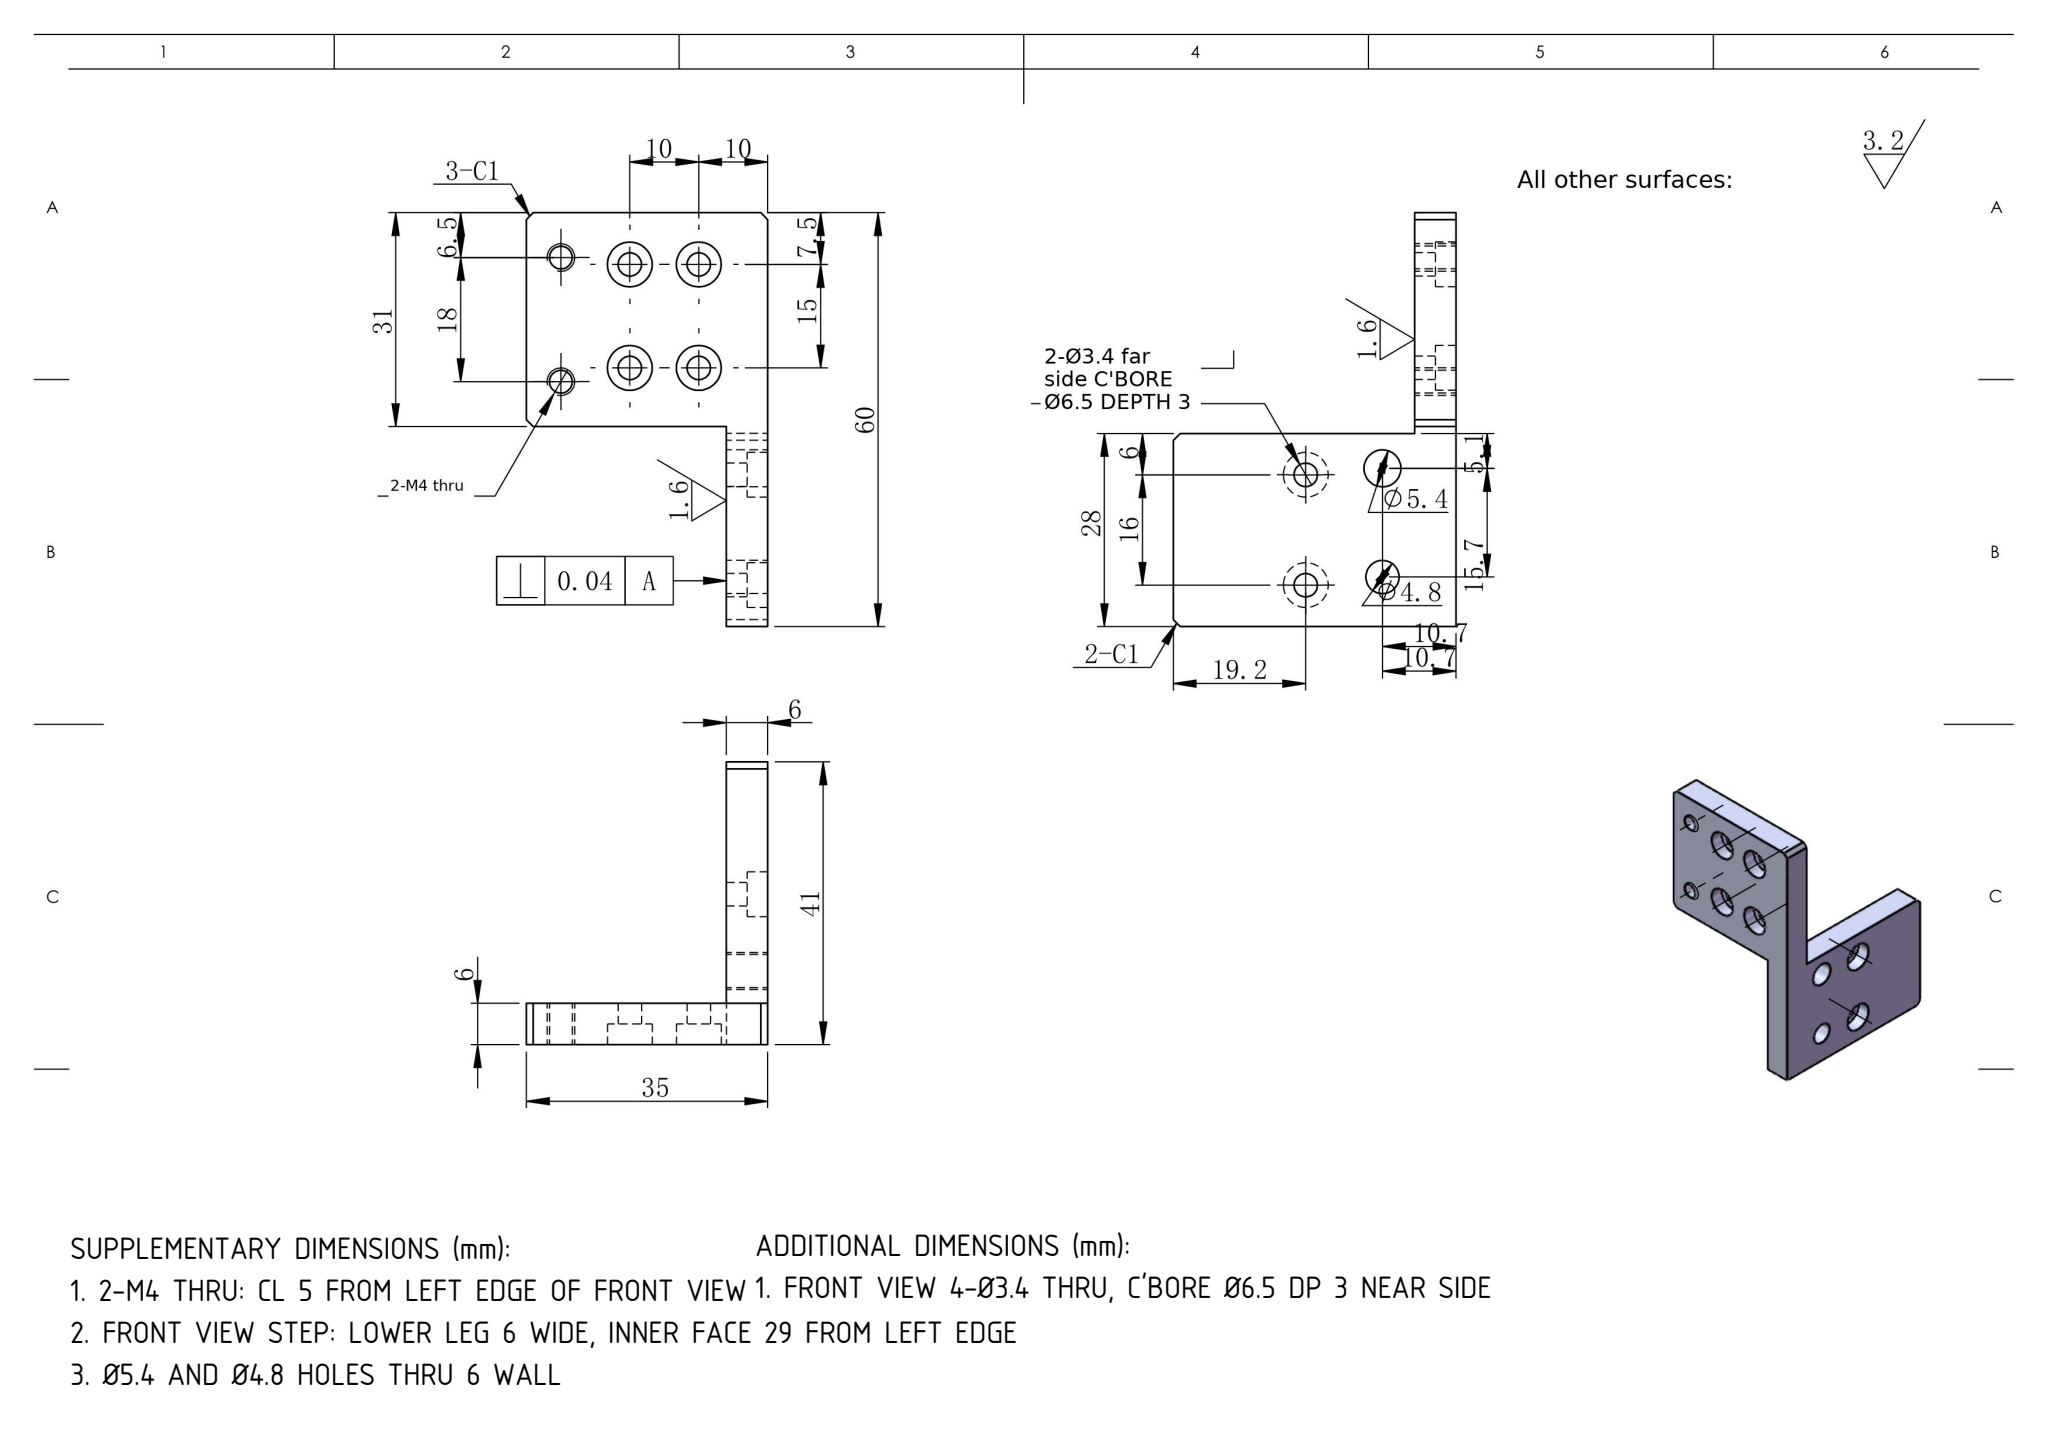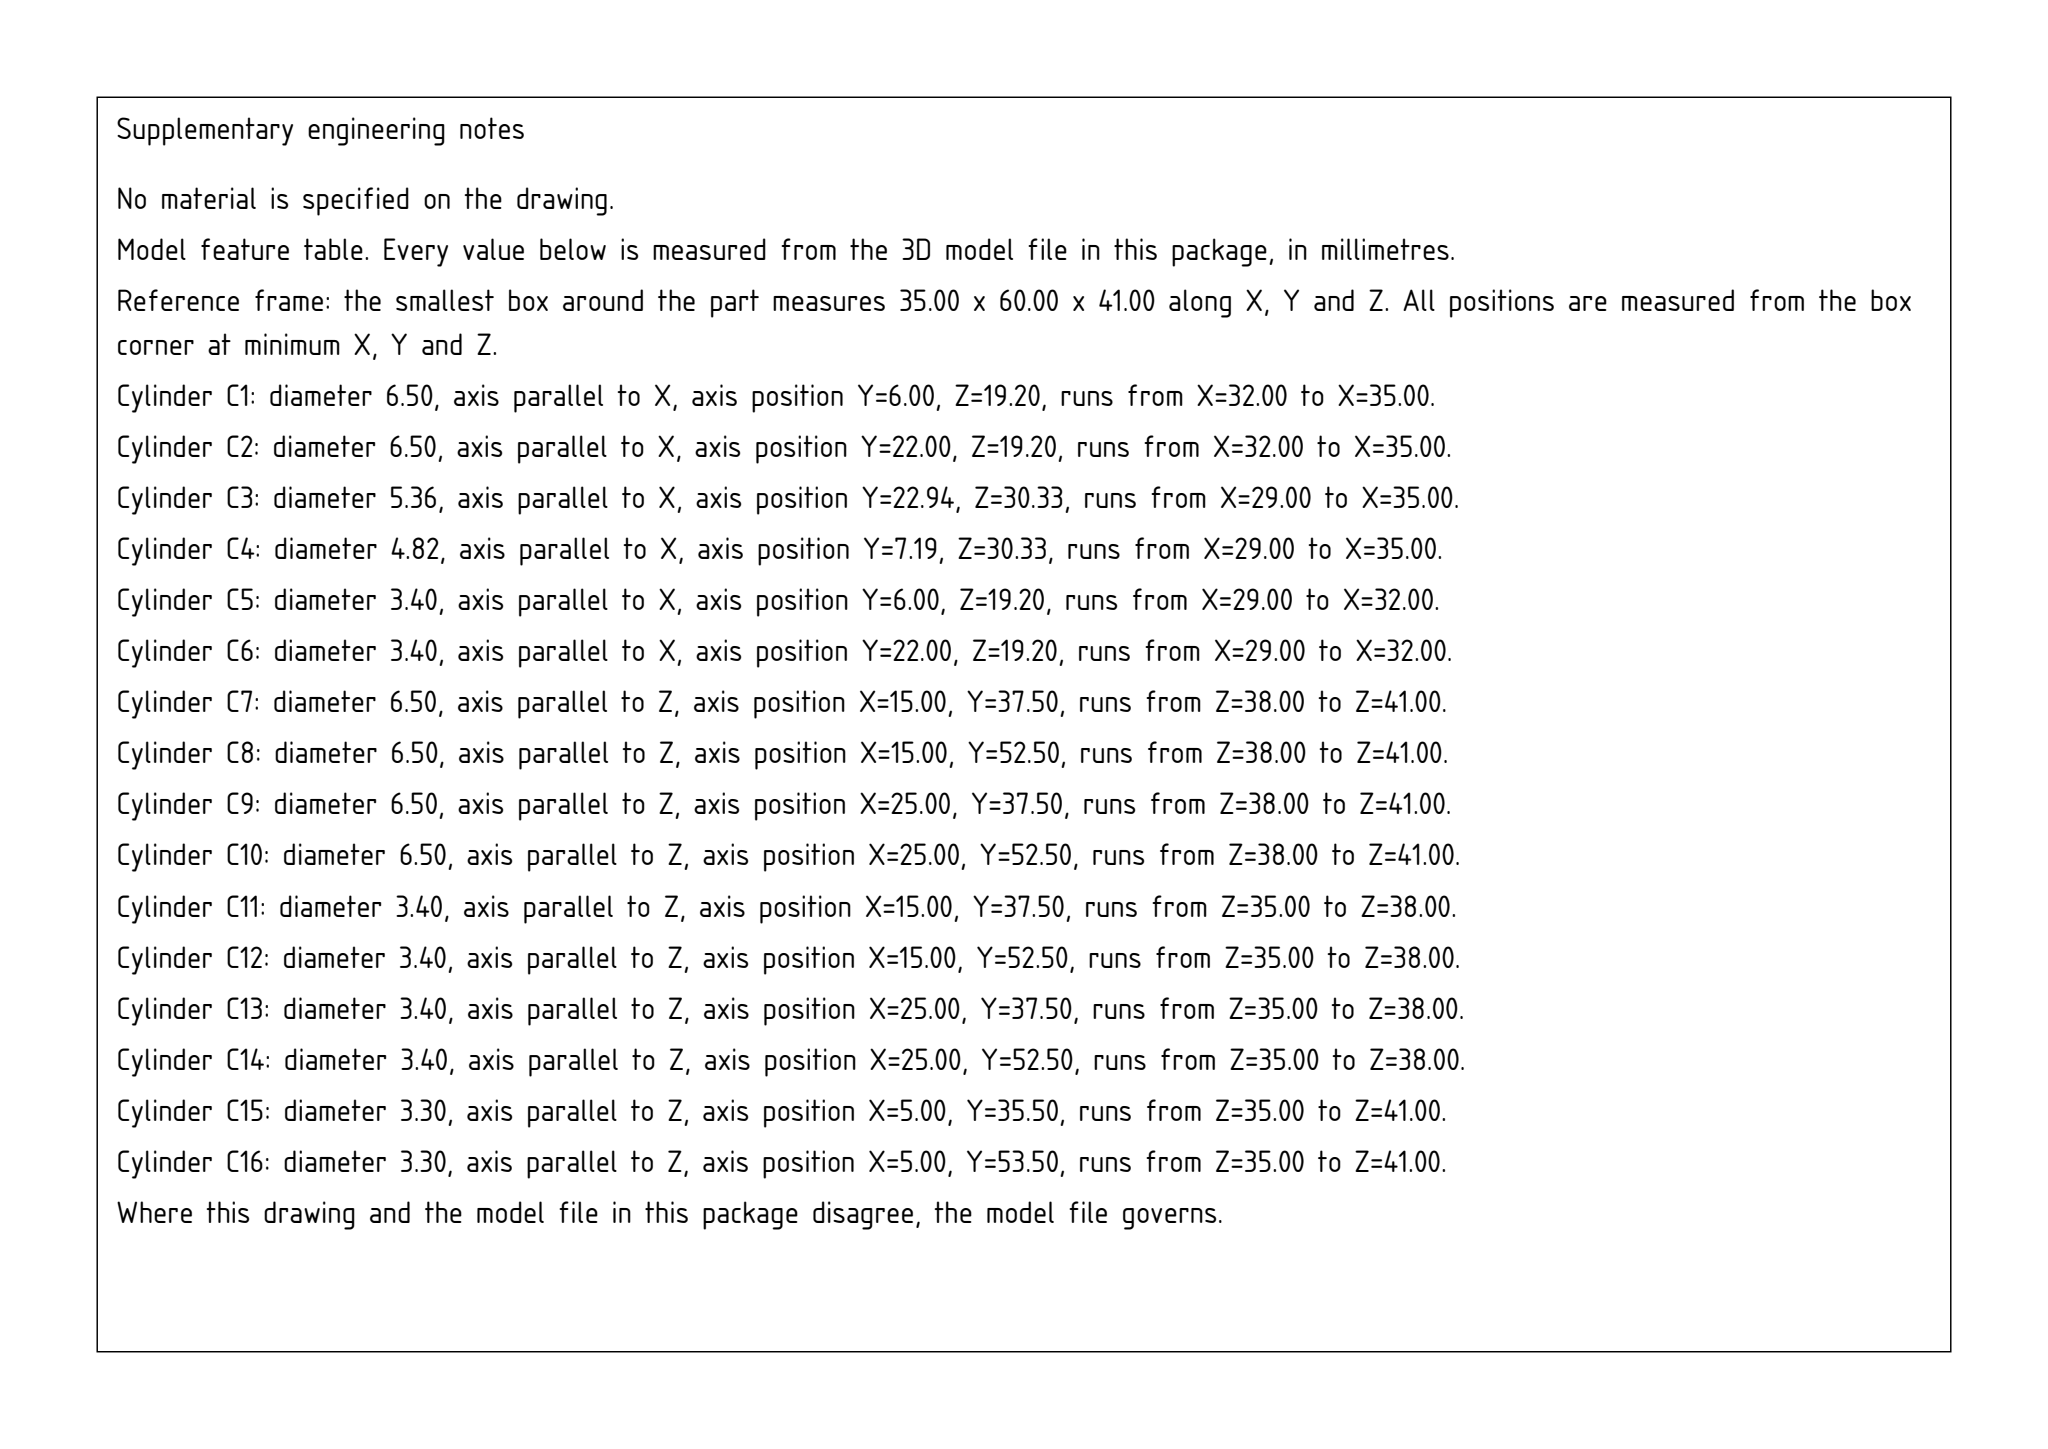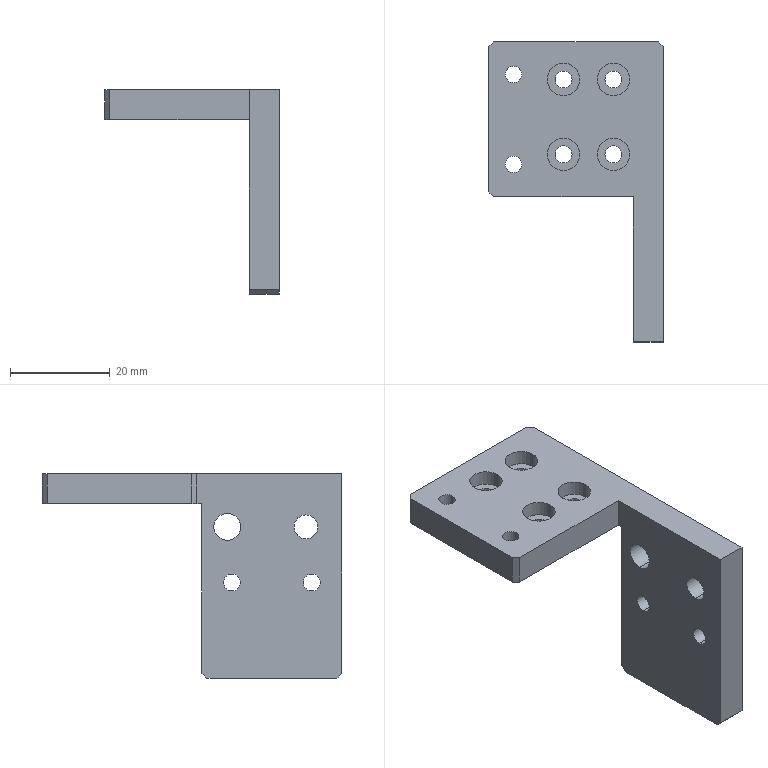Part | SolidWorks | mm | 1 solid | 53 faces | box 35 x 60 x 41 mm | volume 12311 mm3 | cylinder 32 | plane 21 | commonest cylinder face diameters 6.5 x12 3.4 x12 3.3 x4 5.358 x2 4.812 x2
build123d program:
from build123d import *

# Parameters (mm, degrees)
SKETCH1_W                                       = 35
SKETCH1_H                                       = 60
EXTRUDE1_DEPTH                                  = 6
M3_HEX_SOCKET_HEAD_CAP_SCREW_CBORE1_D           = 3.4
M3_HEX_SOCKET_HEAD_CAP_SCREW_CBORE1_CBORE_D     = 6.5
M3_HEX_SOCKET_HEAD_CAP_SCREW_CBORE1_CBORE_DEPTH = 3
SKETCH5_W                                       = 6
SKETCH5_H                                       = 28
EXTRUDE2_DEPTH                                  = 35
SKETCH6_W                                       = 29
SKETCH6_H                                       = 29
CUT_EXTRUDE1_DEPTH                              = 78.782
CHAMFER1_SIZE                                   = 1
M4_TAPPED_HOLE1_D                               = 3.3
M3_HEX_SOCKET_HEAD_CAP_SCREW_CBORE2_D           = 3.4
M3_HEX_SOCKET_HEAD_CAP_SCREW_CBORE2_CBORE_D     = 6.5
M3_HEX_SOCKET_HEAD_CAP_SCREW_CBORE2_CBORE_DEPTH = 3
CHAMFER2_SIZE                                   = 1
SKETCH11_R                                      = 2.679
SKETCH11_R_2                                    = 2.406
CUT_EXTRUDE2_DEPTH                              = 10


with BuildPart() as part:
    # Sketch1 → Extrude1 (new body)
    with BuildSketch(Plane.XY):
        with Locations((17.5, 30)):
            Rectangle(SKETCH1_W, SKETCH1_H)
    extrude(amount=EXTRUDE1_DEPTH)

    # M3 Hex Socket Head Cap Screw CBORE1 (through all)
    with Locations(Plane.XY.offset(6)):
        with Locations((15, 52.5), (25, 52.5), (25, 37.5), (15, 37.5)):
            CounterBoreHole(M3_HEX_SOCKET_HEAD_CAP_SCREW_CBORE1_D / 2, M3_HEX_SOCKET_HEAD_CAP_SCREW_CBORE1_CBORE_D / 2, M3_HEX_SOCKET_HEAD_CAP_SCREW_CBORE1_CBORE_DEPTH)

    # Sketch5 → Extrude2 (add)
    with BuildSketch(Plane(origin=(0, 0, 0), x_dir=(-1, 0, 0), z_dir=(0, 0, -1))):
        with Locations((-32, 14)):
            Rectangle(SKETCH5_W, SKETCH5_H)
    extrude(amount=EXTRUDE2_DEPTH)

    # Sketch6 → Cut-Extrude1 (cut, through all)
    with BuildSketch(Plane(origin=(0, 0, 0), x_dir=(-1, 0, 0), z_dir=(0, 0, -1))):
        with Locations((-14.5, 14.5)):
            Rectangle(SKETCH6_W, SKETCH6_H)
    extrude(amount=-CUT_EXTRUDE1_DEPTH, mode=Mode.SUBTRACT)

    # Chamfer1
    chamfer1_edges = [part.edges().sort_by_distance(p)[0] for p in [
        (0, 29, 3),
        (0, 60, 3),
        (35, 60, 3),
    ]]
    chamfer(chamfer1_edges, length=CHAMFER1_SIZE)

    # M4 Tapped Hole1 (through all)
    with Locations(Plane.XY.offset(6)):
        with Locations((5, 53.5), (5, 35.5)):
            Hole(M4_TAPPED_HOLE1_D / 2)

    # M3 Hex Socket Head Cap Screw CBORE2 (through all)
    with Locations(Plane(origin=(35, 0, 0), x_dir=(0, 0, -1), z_dir=(1, 0, 0))):
        with Locations((15.8, 22), (15.8, 6)):
            CounterBoreHole(M3_HEX_SOCKET_HEAD_CAP_SCREW_CBORE2_D / 2, M3_HEX_SOCKET_HEAD_CAP_SCREW_CBORE2_CBORE_D / 2, M3_HEX_SOCKET_HEAD_CAP_SCREW_CBORE2_CBORE_DEPTH)

    # Chamfer2
    chamfer2_edges = [part.edges().sort_by_distance(p)[0] for p in [
        (32, 0, -35),
        (32, 28, -35),
    ]]
    chamfer(chamfer2_edges, length=CHAMFER2_SIZE)

    # Sketch11 → Cut-Extrude2 (cut)
    with BuildSketch(Plane(origin=(35, 0, 0), x_dir=(0, 0, -1), z_dir=(1, 0, 0))):
        with Locations((4.667, 22.939)):
            Circle(SKETCH11_R)
        with Locations((4.667, 7.19)):
            Circle(SKETCH11_R_2)
    extrude(amount=-CUT_EXTRUDE2_DEPTH, mode=Mode.SUBTRACT)


solid = part.part